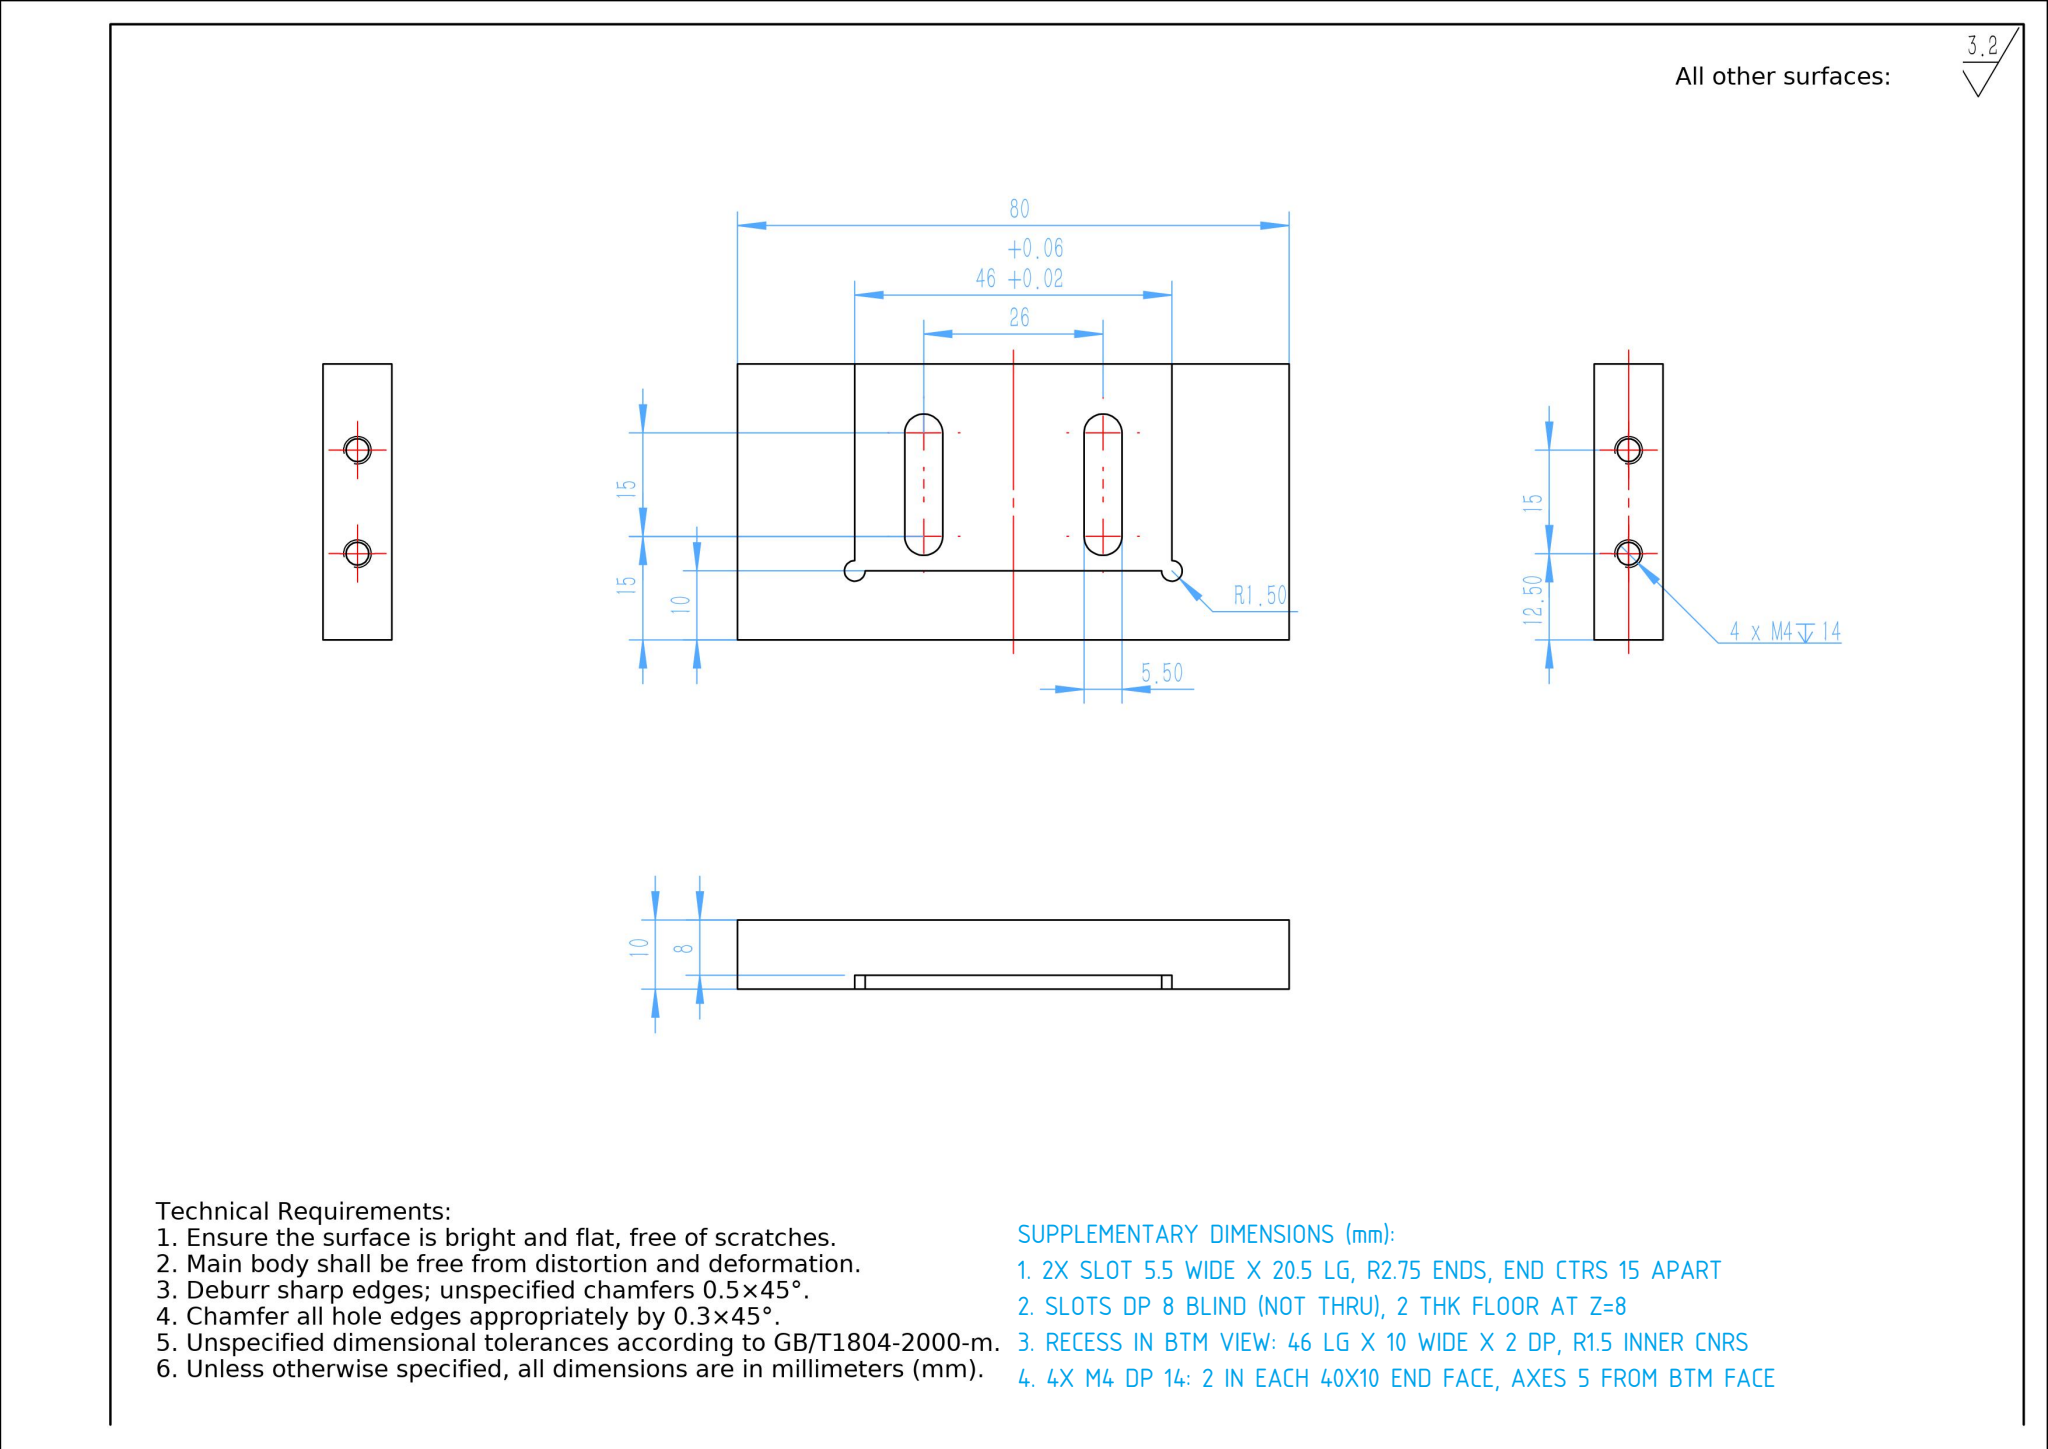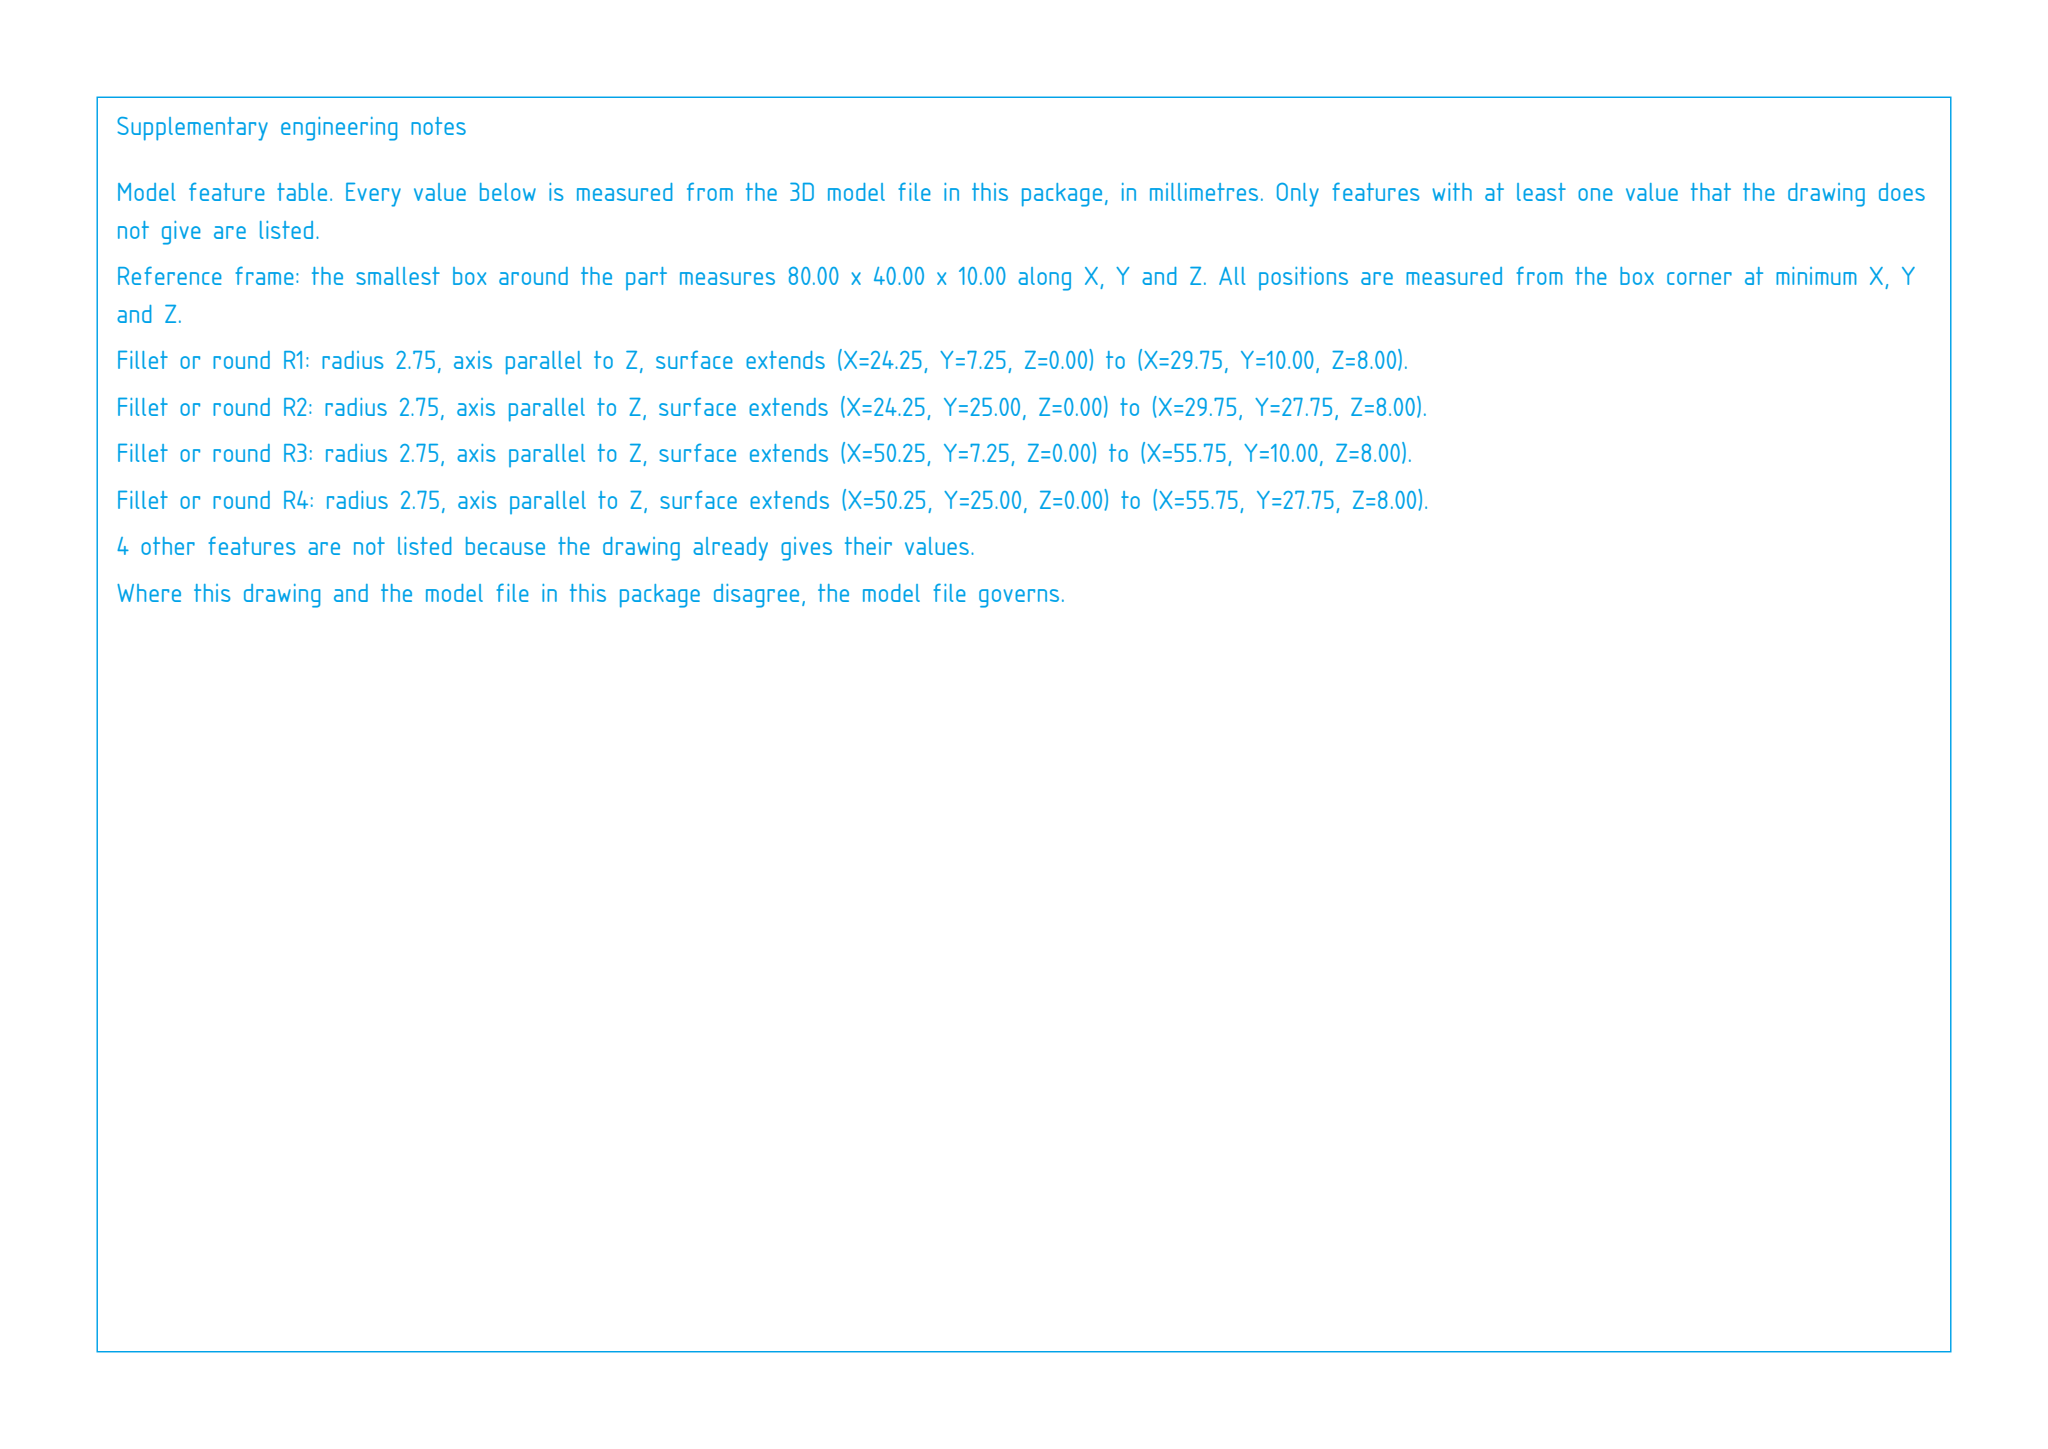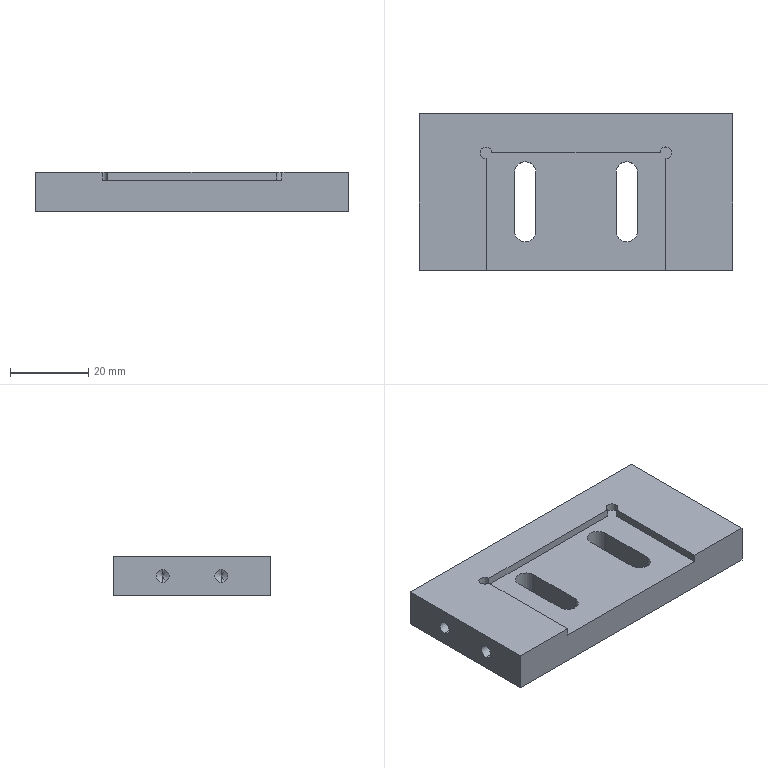Part | SolidWorks | mm | 1 solid | 37 faces | box 80 x 40 x 10 mm | volume 26957 mm3 | cylinder 15 | plane 14 | cone 8 | commonest cylinder face diameters 3.3 x8 5.5 x4 3 x3
build123d program:
from build123d import *

# Parameters (mm, degrees)
SKETCH1_W                  = 80
SKETCH1_H                  = 40
BOSS_EXTRUDE1_DEPTH        = 5
SKETCH2_W                  = 46
SKETCH2_H                  = 30
CUT_EXTRUDE3_DEPTH         = 2
SKETCH4_R                  = 1.5
CUT_EXTRUDE4_DEPTH         = 46.431
CUT_EXTRUDE5_DEPTH         = 46.431
M4_TAPPED_HOLE1_AT_2_COUNT = 2
M4_TAPPED_HOLE1_AT_2_PITCH = 15


with BuildPart() as part:
    # Sketch1 → Boss-Extrude1 (new, symmetric)
    with BuildSketch(Plane.XY):
        Rectangle(SKETCH1_W, SKETCH1_H)
    extrude(amount=BOSS_EXTRUDE1_DEPTH, both=True)

    # Sketch2 → Cut-Extrude3 (cut)
    with BuildSketch(Plane.XY.offset(5)):
        with Locations((0, -5)):
            Rectangle(SKETCH2_W, SKETCH2_H)
    extrude(amount=-CUT_EXTRUDE3_DEPTH, mode=Mode.SUBTRACT)

    # Sketch4 → Cut-Extrude4 (cut, through all)
    with BuildSketch(Plane.XY.offset(3)):
        with Locations((-23, 10)):
            Circle(SKETCH4_R)
        with Locations((23, 10)):
            Circle(SKETCH4_R)
    extrude(amount=CUT_EXTRUDE4_DEPTH, mode=Mode.SUBTRACT)

    # Sketch5 → Cut-Extrude5 (cut, through all)
    with BuildSketch(Plane.XY.offset(3)):
        with BuildLine():
            Line((-10.25, 5), (-10.25, -10))
            ThreePointArc((-10.25, -10), (-13, -12.75), (-15.75, -10))
            Line((-15.75, -10), (-15.75, 5))
            ThreePointArc((-15.75, 5), (-13, 7.75), (-10.25, 5))
        make_face()
        with BuildLine():
            Line((15.75, 5), (15.75, -10))
            ThreePointArc((15.75, -10), (13, -12.75), (10.25, -10))
            Line((10.25, -10), (10.25, 5))
            ThreePointArc((10.25, 5), (13, 7.75), (15.75, 5))
        make_face()
    extrude(amount=-CUT_EXTRUDE5_DEPTH, mode=Mode.SUBTRACT)

    # Sketch6 → M4 Tapped Hole1 (revolve, cut)
    with BuildSketch(Plane(origin=(-40, -7.5, 0), x_dir=(0, 0, 1), z_dir=(0, 1, 0))):
        Polygon((0, 0), (0, 17.091), (1.65, 16.1), (1.65, 0), align=None)
    m4_tapped_hole1 = revolve(axis=Axis((-46.35, -7.5, 0), (1, 0, 0)), mode=Mode.SUBTRACT)

    # M4 Tapped Hole1 at 2: M4 Tapped Hole1 ×2
    with Locations(*[(0, i * M4_TAPPED_HOLE1_AT_2_PITCH, 0) for i in range(1, M4_TAPPED_HOLE1_AT_2_COUNT)]):
        add(m4_tapped_hole1, mode=Mode.SUBTRACT)

    # Mirror1: M4 Tapped Hole1 across plane
    add(m4_tapped_hole1.mirror(Plane(origin=(0, 0, 0), x_dir=(0, 0, 1), z_dir=(1, 0, 0))), mode=Mode.SUBTRACT)

    # Mirror1 copy 1 sketch → Mirror1 copy 1 (revolve, cut)
    with BuildSketch(Plane(origin=(40, 7.5, 0), x_dir=(0, 0, 1), z_dir=(0, 1, 0))):
        Polygon((0, 0), (0, -17.091), (1.65, -16.1), (1.65, 0), align=None)
    revolve(axis=Axis((46.35, 7.5, 0), (1, 0, 0)), mode=Mode.SUBTRACT)


solid = part.part